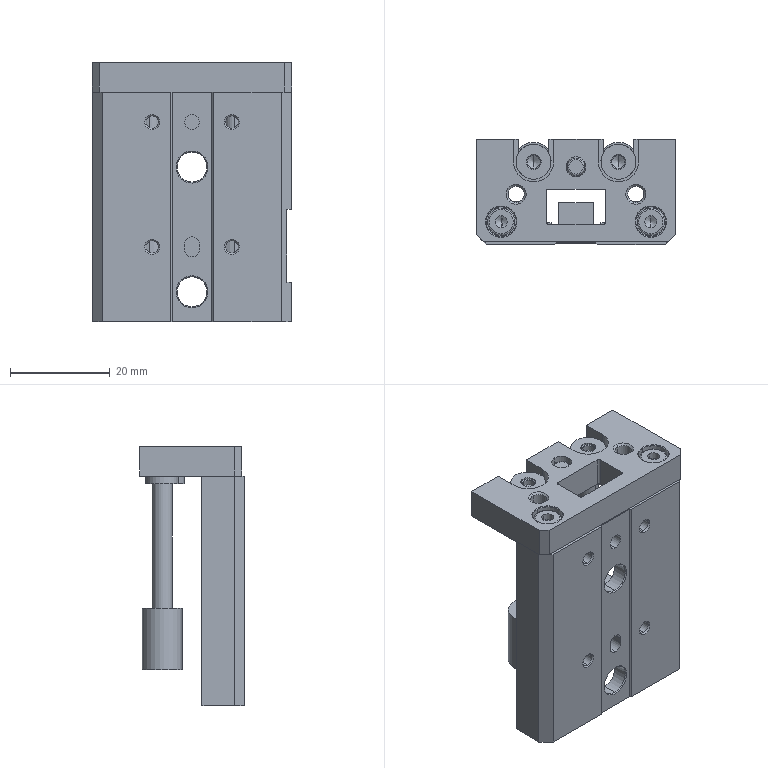Component | SolidWorks | SL010-LeftStreamline-1-1_SL010-SideClampAssembly-DB-1-1_SL010-HLQ8X10SAF(0)+(DS1-H-2)-DB-1-1_SL010-HLQ8X10-S-AF-0-rod-DB-1-1 | 1 solid | 215 faces | box 40 x 21 x 52 mm | volume 17253 mm3 | plane 88 | cylinder 83 | cone 38 | torus 6 | commonest cylinder face diameters 2.459 x12 6 x12 3 x9 5.5 x8 8 x8 7 x6 4 x6 2.4 x4
build123d program:
from build123d import *

# Parameters (mm, degrees)
BOSS_EXTRUDE1_DEPTH     = 2.9
BOSS_EXTRUDE2_DEPTH     = 3.1
BOSS_EXTRUDE3_DEPTH     = 46
BOSS_EXTRUDE4_DEPTH     = 18
CUT_EXTRUDE1_DEPTH      = 4
CUT_EXTRUDE1_DEPTH_BACK = 4
SKETCH13_W              = 14.6
SKETCH13_H              = 1
SKETCH22_W              = 1.5
SKETCH22_H              = 3
CUT_EXTRUDE2_DEPTH      = 2.5


with BuildPart() as part:
    # Sketch1 → Revolve1 (revolve)
    with BuildSketch(Plane.XY, mode=Mode.PRIVATE) as revolve1_sk:
        Polygon((-3.769, 8.5), (-4.6, 9.94), (-5.8, 9.94), (-5.8, 9.8), (-6, 10), (-6.3, 10), (-6.3, 12), (-4.4, 12), (-4.4, 11.25), (-1.5, 11.25), (-1.5, 11.75), (0, 11.75), (0, 10.5), (25, 10.5), (25, 12.5), (37.3, 12.5), (37.3, 8.5), align=None)
    revolve(revolve1_sk.sketch.rotate(Axis((37.3, 8.5, 0), (-1, 0, 0)), 270), axis=Axis((37.3, 8.5, 0), (-1, 0, 0)))

    # Sketch2 → Boss-Extrude1 (add)
    with BuildSketch(Plane(origin=(-4.4, 0, 0), x_dir=(0, 0, -1), z_dir=(1, 0, 0))):
        with BuildLine():
            Line((-16, 18.586), (-16, -18.586))
            Line((-16, -18.586), (-14.586, -20))
            Line((-14.586, -20), (4.5, -20))
            Line((4.5, -20), (4.5, -11.5))
            Line((4.5, -11.5), (0, -11.5))
            ThreePointArc((0, -11.5), (-3, -8.5), (0, -5.5))
            Line((0, -5.5), (4.5, -5.5))
            Line((4.5, -5.5), (4.5, 5.5))
            Line((4.5, 5.5), (0, 5.5))
            ThreePointArc((0, 5.5), (-3, 8.5), (0, 11.5))
            Line((0, 11.5), (4.5, 11.5))
            Line((4.5, 11.5), (4.5, 20))
            Line((4.5, 20), (-14.586, 20))
            Line((-14.586, 20), (-16, 18.586))
        make_face()
        with BuildLine():
            Line((-12.5, 5.5), (-12.5, -5.5))
            ThreePointArc((-12.5, -5.5), (-12.354, -5.854), (-12, -6))
            Line((-12, -6), (-6, -6))
            ThreePointArc((-6, -6), (-5.646, -5.854), (-5.5, -5.5))
            Line((-5.5, -5.5), (-5.5, 5.5))
            ThreePointArc((-5.5, 5.5), (-5.646, 5.854), (-6, 6))
            Line((-6, 6), (-12, 6))
            ThreePointArc((-12, 6), (-12.354, 5.854), (-12.5, 5.5))
        make_face(mode=Mode.SUBTRACT)
    extrude(amount=BOSS_EXTRUDE1_DEPTH)

    # Sketch3 → Boss-Extrude2 (add)
    with BuildSketch(Plane(origin=(-7.5, 0, 0), x_dir=(0, 0, -1), z_dir=(1, 0, 0))):
        with BuildLine():
            Line((-16, 18.586), (-16, -18.586))
            Line((-16, -18.586), (-14.586, -20))
            Line((-14.586, -20), (4.5, -20))
            Line((4.5, -20), (4.5, -12.5))
            Line((4.5, -12.5), (0, -12.5))
            ThreePointArc((0, -12.5), (-4, -8.5), (0, -4.5))
            Line((0, -4.5), (4.5, -4.5))
            Line((4.5, -4.5), (4.5, 4.5))
            Line((4.5, 4.5), (0, 4.5))
            ThreePointArc((0, 4.5), (-4, 8.5), (0, 12.5))
            Line((0, 12.5), (4.5, 12.5))
            Line((4.5, 12.5), (4.5, 20))
            Line((4.5, 20), (-14.586, 20))
            Line((-14.586, 20), (-16, 18.586))
        make_face()
        with BuildLine():
            Line((-12.5, 5.5), (-12.5, -5.5))
            ThreePointArc((-12.5, -5.5), (-12.354, -5.854), (-12, -6))
            Line((-12, -6), (-6, -6))
            ThreePointArc((-6, -6), (-5.646, -5.854), (-5.5, -5.5))
            Line((-5.5, -5.5), (-5.5, 5.5))
            ThreePointArc((-5.5, 5.5), (-5.646, 5.854), (-6, 6))
            Line((-6, 6), (-12, 6))
            ThreePointArc((-12, 6), (-12.354, 5.854), (-12.5, 5.5))
        make_face(mode=Mode.SUBTRACT)
    extrude(amount=BOSS_EXTRUDE2_DEPTH)

    # Sketch4 → Revolve2 (revolve)
    with BuildSketch(Plane.XY, mode=Mode.PRIVATE) as revolve2_sk:
        Polygon((-3.769, -8.5), (-4.6, -7.06), (-5.8, -7.06), (-5.8, -7.2), (-6, -7), (-6.3, -7), (-6.3, -5), (-4.4, -5), (-4.4, -5.75), (-1.5, -5.75), (-1.5, -5.25), (0, -5.25), (0, -6.5), (25, -6.5), (25, -4.5), (37.3, -4.5), (37.3, -8.5), align=None)
    revolve(revolve2_sk.sketch.rotate(Axis((37.3, -8.5, 0), (-1, 0, 0)), 270), axis=Axis((37.3, -8.5, 0), (-1, 0, 0)))

    # Sketch5 → Boss-Extrude3 (add)
    with BuildSketch(Plane(origin=(-1.5, 0, 0), x_dir=(0, 0, -1), z_dir=(1, 0, 0))):
        Polygon((-16.5, 17.92), (-16.5, 4.3), (-16.2, 4), (-16.2, -4), (-16.5, -4.3), (-16.5, -17.95), (-14.5, -19.95), (-8, -19.95), (-8, -9.5), (-12.2, -9.5), (-12.2, -5), (-13.1, -5), (-13.1, 5), (-12.2, 5), (-12.2, 9.5), (-8, 9.5), (-8, 19.92), (-14.5, 19.92), align=None)
    extrude(amount=BOSS_EXTRUDE3_DEPTH)

    # Sketch6 → Boss-Extrude4 (add)
    with BuildSketch(Plane(origin=(17, 0, 0), x_dir=(0, 0, -1), z_dir=(1, 0, 0))):
        Polygon((-13.1, 3), (-13.1, -3), (-13, -3), (-12.5, -3.5), (-8.2, -3.5), (-8.2, 3.5), (-12.5, 3.5), (-13, 3), align=None)
    extrude(amount=BOSS_EXTRUDE4_DEPTH)

    # Sketch7 → Cut-Revolve1 (revolve, cut)
    with BuildSketch(Plane.XY.offset(6.5), mode=Mode.PRIVATE) as cut_revolve1_sk:
        Polygon((-7.5, 12), (-7.5, 14), (-7.121, 13.621), (-1.5, 13.621), (-1.5, 12), align=None)
    revolve(cut_revolve1_sk.sketch.rotate(Axis((-1.5, 12, 6.5), (-1, 0, 0)), 270), axis=Axis((-1.5, 12, 6.5), (-1, 0, 0)), mode=Mode.SUBTRACT)

    # Sketch8 → Cut-Revolve2 (revolve, cut)
    with BuildSketch(Plane.XY.offset(6.5), mode=Mode.PRIVATE) as cut_revolve2_sk:
        Polygon((-7.5, -12), (-7.5, -10), (-7.121, -10.379), (-1.5, -10.379), (-1.5, -12), align=None)
    revolve(cut_revolve2_sk.sketch.rotate(Axis((-1.5, -12, 6.5), (-1, 0, 0)), 270), axis=Axis((-1.5, -12, 6.5), (-1, 0, 0)), mode=Mode.SUBTRACT)

    # Sketch9 → Cut-Revolve3 (revolve, cut)
    with BuildSketch(Plane(origin=(0, 0, 0), x_dir=(1, 0, 0), z_dir=(0, 1, 0)), mode=Mode.PRIVATE) as cut_revolve3_sk:
        Polygon((-7.5, -1), (-7.5, 1), (-2.5, 1), (-2.5, 0.5), (-1.5, 0.5), (-1.5, -1), align=None)
    revolve(cut_revolve3_sk.sketch.rotate(Axis((-1.5, 0, 1), (-1, 0, 0)), 180), axis=Axis((-1.5, 0, 1), (-1, 0, 0)), mode=Mode.SUBTRACT)

    # Sketch10 → Revolve3 (revolve)
    with BuildSketch(Plane(origin=(0, 0, 0), x_dir=(1, 0, 0), z_dir=(0, 1, 0)), mode=Mode.PRIVATE) as revolve3_sk:
        with BuildLine():
            Line((-6.5, -1), (-6.5, 0.45))
            ThreePointArc((-6.5, 0.45), (-6.412, 0.6621), (-6.2, 0.75))
            Line((-6.2, 0.75), (-5.27, 0.75))
            Line((-5.27, 0.75), (-3.5, 1.5))
            Line((-3.5, 1.5), (-3, 1.5))
            Line((-3, 1.5), (-3, 1))
            Line((-3, 1), (-1.5, 1))
            Line((-1.5, 1), (-1.5, 2.5))
            Line((-1.5, 2.5), (0, 2.5))
            Line((0, 2.5), (0, -1))
            Line((0, -1), (-6.5, -1))
        make_face()
    revolve(revolve3_sk.sketch.rotate(Axis((0, 0, 1), (-1, 0, 0)), 180), axis=Axis((0, 0, 1), (-1, 0, 0)))

    # Sketch11 → Cut-Revolve4 (revolve, cut)
    with BuildSketch(Plane.XY.offset(12), mode=Mode.PRIVATE) as cut_revolve4_sk:
        with BuildLine():
            Line((-7.5, 15), (-7.5, 18.141))
            Line((-7.5, 18.141), (-7.359, 18))
            Line((-7.359, 18), (-2.9, 18))
            Line((-2.9, 18), (-2.9, 17.75))
            Line((-2.9, 17.75), (-6.57, 17.75))
            ThreePointArc((-6.57, 17.75), (-6.803, 17.653), (-6.9, 17.42))
            Line((-6.9, 17.42), (-6.9, 16.2))
            Line((-6.9, 16.2), (-5.5, 16.2))
            Line((-5.5, 16.2), (-4.807, 15))
            Line((-4.807, 15), (-7.5, 15))
        make_face()
    revolve(cut_revolve4_sk.sketch.rotate(Axis((-4.807, 15, 12), (-1, 0, 0)), 270), axis=Axis((-4.807, 15, 12), (-1, 0, 0)), mode=Mode.SUBTRACT)

    # Sketch12 → Cut-Revolve5 (revolve, cut)
    with BuildSketch(Plane.XY.offset(12), mode=Mode.PRIVATE) as cut_revolve5_sk:
        with BuildLine():
            Line((-7.5, -15), (-7.5, -11.859))
            Line((-7.5, -11.859), (-7.359, -12))
            Line((-7.359, -12), (-2.9, -12))
            Line((-2.9, -12), (-2.9, -12.25))
            Line((-2.9, -12.25), (-6.57, -12.25))
            ThreePointArc((-6.57, -12.25), (-6.803, -12.347), (-6.9, -12.58))
            Line((-6.9, -12.58), (-6.9, -13.8))
            Line((-6.9, -13.8), (-5.5, -13.8))
            Line((-5.5, -13.8), (-4.807, -15))
            Line((-4.807, -15), (-7.5, -15))
        make_face()
    revolve(cut_revolve5_sk.sketch.rotate(Axis((-4.807, -15, 12), (-1, 0, 0)), 270), axis=Axis((-4.807, -15, 12), (-1, 0, 0)), mode=Mode.SUBTRACT)

    # Sketch13 → Cut-Extrude1 (cut, two sides: drawn at the far end of the back side and taken through both)
    with BuildSketch(Plane.XY.offset(12).offset(-CUT_EXTRUDE1_DEPTH_BACK)):
        with Locations((29.3, 19.5)):
            Rectangle(SKETCH13_W, SKETCH13_H)
    extrude(amount=CUT_EXTRUDE1_DEPTH + CUT_EXTRUDE1_DEPTH_BACK, mode=Mode.SUBTRACT)

    # Sketch14 → Cut-Revolve6 (revolve, cut)
    with BuildSketch(Plane.XY.offset(12), mode=Mode.PRIVATE) as cut_revolve6_sk:
        Polygon((25.8, 16), (24.57, 16), (24.57, 18.73), (24.3, 19), (25.8, 19), align=None)
    revolve(cut_revolve6_sk.sketch.rotate(Axis((25.8, 19, 12), (0, -1, 0)), 180), axis=Axis((25.8, 19, 12), (0, -1, 0)), mode=Mode.SUBTRACT)

    # Sketch15 → Cut-Revolve7 (revolve, cut)
    with BuildSketch(Plane.XY.offset(12), mode=Mode.PRIVATE) as cut_revolve7_sk:
        Polygon((32.8, 16), (31.57, 16), (31.57, 18.73), (31.3, 19), (32.8, 19), align=None)
    revolve(cut_revolve7_sk.sketch.rotate(Axis((32.8, 19, 12), (0, -1, 0)), 90), axis=Axis((32.8, 19, 12), (0, -1, 0)), mode=Mode.SUBTRACT)

    # Sketch16 → Cut-Revolve8 (revolve, cut)
    with BuildSketch(Plane(origin=(0, 0, 0), x_dir=(1, 0, 0), z_dir=(0, 1, 0)), mode=Mode.PRIVATE) as cut_revolve8_sk:
        Polygon((13.5, -16.2), (10.288, -16.2), (10.5, -15.988), (10.5, -13), (13.5, -13), align=None)
    revolve(cut_revolve8_sk.sketch.rotate(Axis((13.5, 0, 13), (0, 0, 1)), 180), axis=Axis((13.5, 0, 13), (0, 0, 1)), mode=Mode.SUBTRACT)

    # Sketch17 → Cut-Revolve9 (revolve, cut)
    with BuildSketch(Plane(origin=(0, 0, 0), x_dir=(1, 0, 0), z_dir=(0, 1, 0)), mode=Mode.PRIVATE) as cut_revolve9_sk:
        Polygon((38.5, -16.2), (35.288, -16.2), (35.5, -15.988), (35.5, -13.1), (38.5, -13.1), align=None)
    revolve(cut_revolve9_sk.sketch.rotate(Axis((38.5, 0, 13.1), (0, 0, 1)), 180), axis=Axis((38.5, 0, 13.1), (0, 0, 1)), mode=Mode.SUBTRACT)

    # Sketch18 → Cut-Revolve10 (revolve, cut)
    with BuildSketch(Plane(origin=(0, 8, 0), x_dir=(1, 0, 0), z_dir=(0, 1, 0)), mode=Mode.PRIVATE) as cut_revolve10_sk:
        Polygon((4.5, -16.5), (3, -16.5), (3.271, -16.23), (3.271, -12.2), (4.5, -12.2), align=None)
    revolve(cut_revolve10_sk.sketch.rotate(Axis((4.5, 8, 12.2), (0, 0, 1)), 180), axis=Axis((4.5, 8, 12.2), (0, 0, 1)), mode=Mode.SUBTRACT)

    # Sketch19 → Cut-Revolve11 (revolve, cut)
    with BuildSketch(Plane(origin=(0, 8, 0), x_dir=(1, 0, 0), z_dir=(0, 1, 0)), mode=Mode.PRIVATE) as cut_revolve11_sk:
        Polygon((29.5, -16.5), (28, -16.5), (28.27, -16.23), (28.27, -12.2), (29.5, -12.2), align=None)
    revolve(cut_revolve11_sk.sketch.rotate(Axis((29.5, 8, 12.2), (0, 0, 1)), 180), axis=Axis((29.5, 8, 12.2), (0, 0, 1)), mode=Mode.SUBTRACT)

    # Sketch20 → Cut-Revolve12 (revolve, cut)
    with BuildSketch(Plane(origin=(0, -8, 0), x_dir=(1, 0, 0), z_dir=(0, 1, 0)), mode=Mode.PRIVATE) as cut_revolve12_sk:
        Polygon((4.5, -16.5), (3, -16.5), (3.271, -16.23), (3.271, -12.2), (4.5, -12.2), align=None)
    revolve(cut_revolve12_sk.sketch.rotate(Axis((4.5, -8, 12.2), (0, 0, 1)), 180), axis=Axis((4.5, -8, 12.2), (0, 0, 1)), mode=Mode.SUBTRACT)

    # Sketch21 → Cut-Revolve13 (revolve, cut)
    with BuildSketch(Plane(origin=(0, -8, 0), x_dir=(1, 0, 0), z_dir=(0, 1, 0)), mode=Mode.PRIVATE) as cut_revolve13_sk:
        Polygon((29.5, -16.5), (28, -16.5), (28.27, -16.23), (28.27, -12.2), (29.5, -12.2), align=None)
    revolve(cut_revolve13_sk.sketch.rotate(Axis((29.5, -8, 12.2), (0, 0, 1)), 180), axis=Axis((29.5, -8, 12.2), (0, 0, 1)), mode=Mode.SUBTRACT)

    # Sketch22 → Cut-Revolve14 (revolve, cut)
    with BuildSketch(Plane(origin=(0, 0, 0), x_dir=(1, 0, 0), z_dir=(0, 1, 0)), mode=Mode.PRIVATE) as cut_revolve14_sk:
        with Locations((5.25, -14.7)):
            Rectangle(SKETCH22_W, SKETCH22_H)
    revolve(cut_revolve14_sk.sketch.rotate(Axis((4.5, 0, 16.2), (0, 0, -1)), 180), axis=Axis((4.5, 0, 16.2), (0, 0, -1)), mode=Mode.SUBTRACT)

    # Sketch23 → Cut-Extrude2 (cut)
    with BuildSketch(Plane.XY.offset(16.2)):
        with BuildLine():
            Line((29, -1.5), (30, -1.5))
            ThreePointArc((30, -1.5), (31.061, -1.061), (31.5, 0))
            ThreePointArc((31.5, 0), (31.061, 1.061), (30, 1.5))
            Line((30, 1.5), (29, 1.5))
            ThreePointArc((29, 1.5), (27.939, 1.061), (27.5, 0))
            ThreePointArc((27.5, 0), (27.939, -1.061), (29, -1.5))
        make_face()
    extrude(amount=-CUT_EXTRUDE2_DEPTH, mode=Mode.SUBTRACT)


solid = part.part

# Placed as in the assembly
solid = solid.moved(Location((-633.5, -115.904, -665.535), (90, 0, -90)))